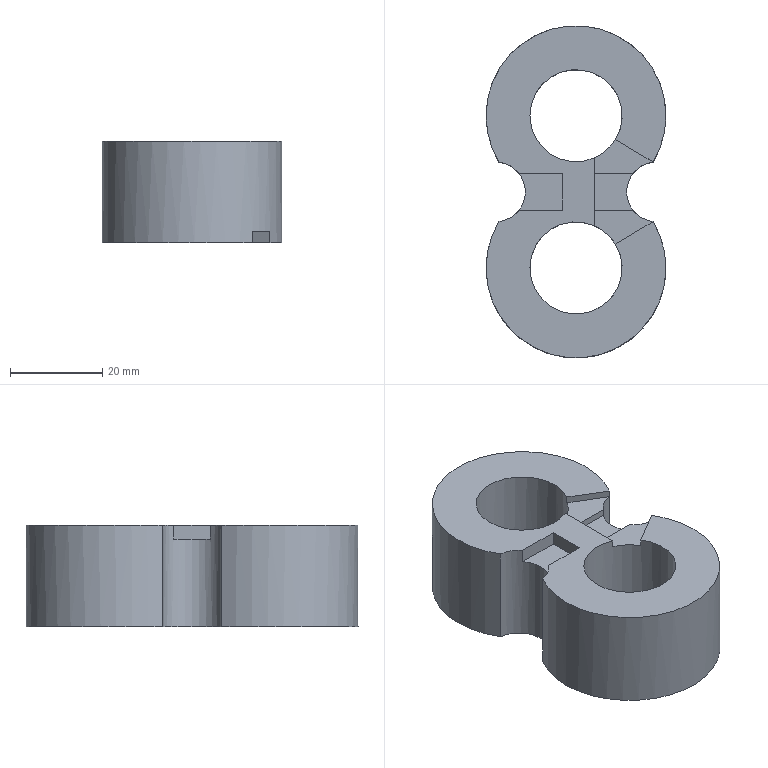Component | NX | 5_2 | 1 solid | 36 faces | volume 34012 mm3 | plane 20 | cylinder 16 | commonest cylinder face diameters 13 x2 39 x2 20 x2 2 x2 32 x2 5 x2 24 x2 1 x1